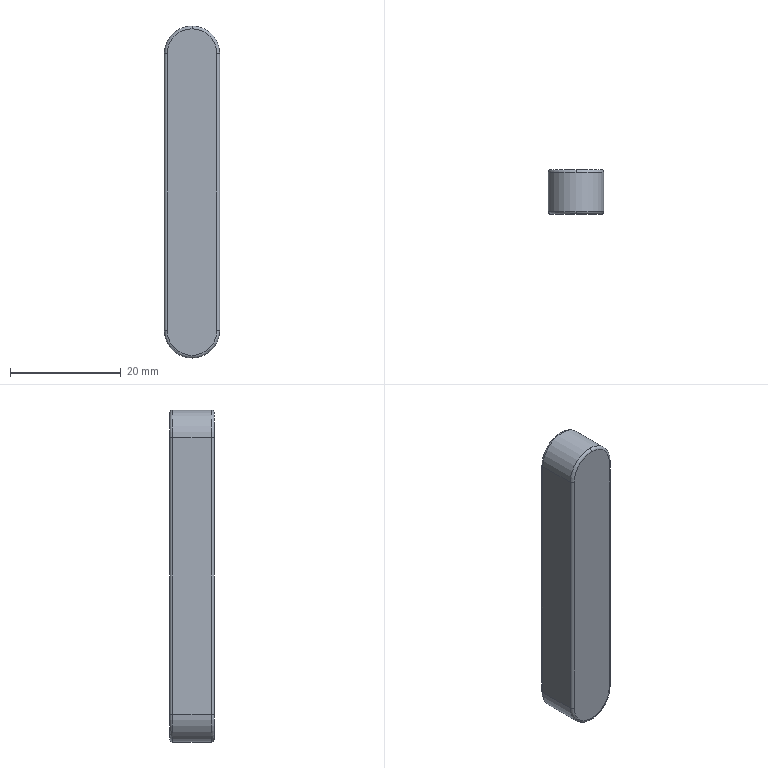Component | SolidWorks | 10X8X50ParallelKey-1 | 1 solid | 17 faces | box 10 x 8 x 60 mm | volume 4614 mm3 | cylinder 7 | torus 6 | plane 4 | commonest cylinder face diameters 1 x4 10 x3 | material AISI 1045 Steel, cold drawn
build123d program:
from build123d import *

# Parameters (mm, degrees)
BOSS_EXTRUDE1_DEPTH = 8
FILLET1_R           = 0.5


with BuildPart() as part:
    # Sketch1 → Boss-Extrude1 (new body)
    with BuildSketch(Plane.XY):
        with BuildLine():
            Line((-25, 5), (25, 5))
            ThreePointArc((25, 5), (30, 0), (25, -5))
            Line((25, -5), (-25, -5))
            ThreePointArc((-25, -5), (-30, 0), (-25, 5))
        make_face()
    extrude(amount=BOSS_EXTRUDE1_DEPTH)

    # Fillet1
    fillet1_edges = [part.edges().sort_by_distance(p)[0] for p in [
        (30, 0, 8),
        (0, 5, 8),
        (-30, 0, 8),
        (0, 5, 0),
        (30, 0, 0),
        (0, -5, 0),
        (-30, 0, 0),
        (0, -5, 8),
    ]]
    fillet(fillet1_edges, radius=FILLET1_R)


solid = part.part

# Placed as in the assembly
solid = solid.moved(Location((0, 18, 0), (90, 0, 90)))
STEP:
#1=CARTESIAN_POINT('',(0.,0.4134,1.181));
#2=VERTEX_POINT('',#1);
#3=CARTESIAN_POINT('',(0.1969,0.4134,0.9843));
#4=VERTEX_POINT('',#3);
#5=CARTESIAN_POINT('',(0.,0.4134,0.9843));
#6=DIRECTION('',(-0.,1.,0.));
#7=DIRECTION('',(0.,-0.,1.));
#8=AXIS2_PLACEMENT_3D('',#5,#6,#7);
#9=CIRCLE('',#8,0.1969);
#10=EDGE_CURVE('',#2,#4,#9,.T.);
#11=ORIENTED_EDGE('',*,*,#10,.F.);
#12=CARTESIAN_POINT('',(0.,0.3937,1.161));
#13=VERTEX_POINT('',#12);
#14=CARTESIAN_POINT('',(0.,0.4134,1.161));
#15=DIRECTION('',(1.,0.,0.));
#16=DIRECTION('',(-0.,1.,0.));
#17=AXIS2_PLACEMENT_3D('',#14,#15,#16);
#18=CIRCLE('',#17,0.01969);
#19=EDGE_CURVE('',#2,#13,#18,.T.);
#20=ORIENTED_EDGE('',*,*,#19,.T.);
#21=CARTESIAN_POINT('',(0.1772,0.3937,0.9843));
#22=VERTEX_POINT('',#21);
#23=CARTESIAN_POINT('',(0.,0.3937,0.9843));
#24=DIRECTION('',(0.,-1.,-0.));
#25=DIRECTION('',(0.,0.,1.));
#26=AXIS2_PLACEMENT_3D('',#23,#24,#25);
#27=CIRCLE('',#26,0.1772);
#28=EDGE_CURVE('',#22,#13,#27,.T.);
#29=ORIENTED_EDGE('',*,*,#28,.F.);
#30=CARTESIAN_POINT('',(0.1772,0.4134,0.9843));
#31=DIRECTION('',(0.,-0.,1.));
#32=DIRECTION('',(0.,1.,0.));
#33=AXIS2_PLACEMENT_3D('',#30,#31,#32);
#34=CIRCLE('',#33,0.01969);
#35=EDGE_CURVE('',#22,#4,#34,.T.);
#36=ORIENTED_EDGE('',*,*,#35,.T.);
#37=EDGE_LOOP('',(#11,#20,#29,#36));
#38=FACE_OUTER_BOUND('',#37,.T.);
#39=CARTESIAN_POINT('',(0.,0.4134,0.9843));
#40=DIRECTION('',(0.,-1.,-0.));
#41=DIRECTION('',(-0.,-0.,1.));
#42=AXIS2_PLACEMENT_3D('',#39,#40,#41);
#43=TOROIDAL_SURFACE('',#42,0.1772,0.01969);
#44=ADVANCED_FACE('',(#38),#43,.T.);
#45=CARTESIAN_POINT('',(0.,0.7087,1.161));
#46=VERTEX_POINT('',#45);
#47=CARTESIAN_POINT('',(0.1772,0.7087,0.9843));
#48=VERTEX_POINT('',#47);
#49=CARTESIAN_POINT('',(0.,0.7087,0.9843));
#50=DIRECTION('',(-0.,1.,0.));
#51=DIRECTION('',(0.,0.,1.));
#52=AXIS2_PLACEMENT_3D('',#49,#50,#51);
#53=CIRCLE('',#52,0.1772);
#54=EDGE_CURVE('',#46,#48,#53,.T.);
#55=ORIENTED_EDGE('',*,*,#54,.F.);
#56=CARTESIAN_POINT('',(0.,0.689,1.181));
#57=VERTEX_POINT('',#56);
#58=CARTESIAN_POINT('',(0.,0.689,1.161));
#59=DIRECTION('',(1.,0.,0.));
#60=DIRECTION('',(-0.,1.,0.));
#61=AXIS2_PLACEMENT_3D('',#58,#59,#60);
#62=CIRCLE('',#61,0.01969);
#63=EDGE_CURVE('',#46,#57,#62,.T.);
#64=ORIENTED_EDGE('',*,*,#63,.T.);
#65=CARTESIAN_POINT('',(0.1969,0.689,0.9843));
#66=VERTEX_POINT('',#65);
#67=CARTESIAN_POINT('',(0.,0.689,0.9843));
#68=DIRECTION('',(0.,-1.,-0.));
#69=DIRECTION('',(0.,0.,1.));
#70=AXIS2_PLACEMENT_3D('',#67,#68,#69);
#71=CIRCLE('',#70,0.1969);
#72=EDGE_CURVE('',#66,#57,#71,.T.);
#73=ORIENTED_EDGE('',*,*,#72,.F.);
#74=CARTESIAN_POINT('',(0.1772,0.689,0.9843));
#75=DIRECTION('',(0.,-0.,1.));
#76=DIRECTION('',(0.,1.,0.));
#77=AXIS2_PLACEMENT_3D('',#74,#75,#76);
#78=CIRCLE('',#77,0.01969);
#79=EDGE_CURVE('',#66,#48,#78,.T.);
#80=ORIENTED_EDGE('',*,*,#79,.T.);
#81=EDGE_LOOP('',(#55,#64,#73,#80));
#82=FACE_OUTER_BOUND('',#81,.T.);
#83=CARTESIAN_POINT('',(0.,0.689,0.9843));
#84=DIRECTION('',(0.,-1.,-0.));
#85=DIRECTION('',(0.,-0.,1.));
#86=AXIS2_PLACEMENT_3D('',#83,#84,#85);
#87=TOROIDAL_SURFACE('',#86,0.1772,0.01969);
#88=ADVANCED_FACE('',(#82),#87,.T.);
#89=CARTESIAN_POINT('',(0.1969,0.4134,-0.9843));
#90=VERTEX_POINT('',#89);
#91=CARTESIAN_POINT('',(0.,0.4134,-1.181));
#92=VERTEX_POINT('',#91);
#93=CARTESIAN_POINT('',(0.,0.4134,-0.9843));
#94=DIRECTION('',(-0.,1.,0.));
#95=DIRECTION('',(-0.,-0.,1.));
#96=AXIS2_PLACEMENT_3D('',#93,#94,#95);
#97=CIRCLE('',#96,0.1969);
#98=EDGE_CURVE('',#90,#92,#97,.T.);
#99=ORIENTED_EDGE('',*,*,#98,.T.);
#100=CARTESIAN_POINT('',(0.,0.689,-1.181));
#101=VERTEX_POINT('',#100);
#102=CARTESIAN_POINT('',(0.,0.3937,-1.181));
#103=DIRECTION('',(-0.,1.,0.));
#104=VECTOR('',#103,39.37);
#105=LINE('',#102,#104);
#106=EDGE_CURVE('',#92,#101,#105,.T.);
#107=ORIENTED_EDGE('',*,*,#106,.T.);
#108=CARTESIAN_POINT('',(0.1969,0.689,-0.9843));
#109=VERTEX_POINT('',#108);
#110=CARTESIAN_POINT('',(0.,0.689,-0.9843));
#111=DIRECTION('',(0.,-1.,-0.));
#112=DIRECTION('',(0.,0.,1.));
#113=AXIS2_PLACEMENT_3D('',#110,#111,#112);
#114=CIRCLE('',#113,0.1969);
#115=EDGE_CURVE('',#101,#109,#114,.T.);
#116=ORIENTED_EDGE('',*,*,#115,.T.);
#117=CARTESIAN_POINT('',(0.1969,0.3937,-0.9843));
#118=DIRECTION('',(-0.,1.,0.));
#119=VECTOR('',#118,39.37);
#120=LINE('',#117,#119);
#121=EDGE_CURVE('',#90,#109,#120,.T.);
#122=ORIENTED_EDGE('',*,*,#121,.F.);
#123=EDGE_LOOP('',(#99,#107,#116,#122));
#124=FACE_OUTER_BOUND('',#123,.T.);
#125=CARTESIAN_POINT('',(0.,0.3937,-0.9843));
#126=DIRECTION('',(-0.,1.,0.));
#127=DIRECTION('',(0.,0.,-1.));
#128=AXIS2_PLACEMENT_3D('',#125,#126,#127);
#129=CYLINDRICAL_SURFACE('',#128,0.1969);
#130=ADVANCED_FACE('',(#124),#129,.T.);
#131=ORIENTED_EDGE('',*,*,#106,.F.);
#132=CARTESIAN_POINT('',(-0.1969,0.4134,-0.9843));
#133=VERTEX_POINT('',#132);
#134=CARTESIAN_POINT('',(0.,0.4134,-0.9843));
#135=DIRECTION('',(-0.,1.,0.));
#136=DIRECTION('',(0.,-0.,1.));
#137=AXIS2_PLACEMENT_3D('',#134,#135,#136);
#138=CIRCLE('',#137,0.1969);
#139=EDGE_CURVE('',#92,#133,#138,.T.);
#140=ORIENTED_EDGE('',*,*,#139,.T.);
#141=CARTESIAN_POINT('',(-0.1969,0.689,-0.9843));
#142=VERTEX_POINT('',#141);
#143=CARTESIAN_POINT('',(-0.1969,0.3937,-0.9843));
#144=DIRECTION('',(-0.,1.,0.));
#145=VECTOR('',#144,39.37);
#146=LINE('',#143,#145);
#147=EDGE_CURVE('',#133,#142,#146,.T.);
#148=ORIENTED_EDGE('',*,*,#147,.T.);
#149=CARTESIAN_POINT('',(0.,0.689,-0.9843));
#150=DIRECTION('',(0.,-1.,-0.));
#151=DIRECTION('',(0.,0.,1.));
#152=AXIS2_PLACEMENT_3D('',#149,#150,#151);
#153=CIRCLE('',#152,0.1969);
#154=EDGE_CURVE('',#142,#101,#153,.T.);
#155=ORIENTED_EDGE('',*,*,#154,.T.);
#156=EDGE_LOOP('',(#131,#140,#148,#155));
#157=FACE_OUTER_BOUND('',#156,.T.);
#158=CARTESIAN_POINT('',(0.,0.3937,-0.9843));
#159=DIRECTION('',(-0.,1.,0.));
#160=DIRECTION('',(0.,0.,-1.));
#161=AXIS2_PLACEMENT_3D('',#158,#159,#160);
#162=CYLINDRICAL_SURFACE('',#161,0.1969);
#163=ADVANCED_FACE('',(#157),#162,.T.);
#164=ORIENTED_EDGE('',*,*,#121,.T.);
#165=CARTESIAN_POINT('',(0.1969,0.689,-0.9843));
#166=DIRECTION('',(0.,-0.,1.));
#167=VECTOR('',#166,39.37);
#168=LINE('',#165,#167);
#169=EDGE_CURVE('',#109,#66,#168,.T.);
#170=ORIENTED_EDGE('',*,*,#169,.T.);
#171=CARTESIAN_POINT('',(0.1969,0.3937,0.9843));
#172=DIRECTION('',(-0.,1.,0.));
#173=VECTOR('',#172,39.37);
#174=LINE('',#171,#173);
#175=EDGE_CURVE('',#4,#66,#174,.T.);
#176=ORIENTED_EDGE('',*,*,#175,.F.);
#177=CARTESIAN_POINT('',(0.1969,0.4134,-0.9843));
#178=DIRECTION('',(0.,0.,-1.));
#179=VECTOR('',#178,39.37);
#180=LINE('',#177,#179);
#181=EDGE_CURVE('',#4,#90,#180,.T.);
#182=ORIENTED_EDGE('',*,*,#181,.T.);
#183=EDGE_LOOP('',(#164,#170,#176,#182));
#184=FACE_OUTER_BOUND('',#183,.T.);
#185=CARTESIAN_POINT('',(0.1969,0.3937,-0.9843));
#186=DIRECTION('',(-1.,-0.,0.));
#187=DIRECTION('',(0.,-1.,-0.));
#188=AXIS2_PLACEMENT_3D('',#185,#186,#187);
#189=PLANE('',#188);
#190=ADVANCED_FACE('',(#184),#189,.F.);
#191=ORIENTED_EDGE('',*,*,#175,.T.);
#192=ORIENTED_EDGE('',*,*,#72,.T.);
#193=CARTESIAN_POINT('',(-0.1969,0.689,0.9843));
#194=VERTEX_POINT('',#193);
#195=CARTESIAN_POINT('',(0.,0.689,0.9843));
#196=DIRECTION('',(0.,-1.,-0.));
#197=DIRECTION('',(0.,0.,1.));
#198=AXIS2_PLACEMENT_3D('',#195,#196,#197);
#199=CIRCLE('',#198,0.1969);
#200=EDGE_CURVE('',#57,#194,#199,.T.);
#201=ORIENTED_EDGE('',*,*,#200,.T.);
#202=CARTESIAN_POINT('',(-0.1969,0.4134,0.9843));
#203=VERTEX_POINT('',#202);
#204=CARTESIAN_POINT('',(-0.1969,0.3937,0.9843));
#205=DIRECTION('',(-0.,1.,0.));
#206=VECTOR('',#205,39.37);
#207=LINE('',#204,#206);
#208=EDGE_CURVE('',#203,#194,#207,.T.);
#209=ORIENTED_EDGE('',*,*,#208,.F.);
#210=CARTESIAN_POINT('',(0.,0.4134,0.9843));
#211=DIRECTION('',(-0.,1.,0.));
#212=DIRECTION('',(-0.,-0.,1.));
#213=AXIS2_PLACEMENT_3D('',#210,#211,#212);
#214=CIRCLE('',#213,0.1969);
#215=EDGE_CURVE('',#203,#2,#214,.T.);
#216=ORIENTED_EDGE('',*,*,#215,.T.);
#217=ORIENTED_EDGE('',*,*,#10,.T.);
#218=EDGE_LOOP('',(#191,#192,#201,#209,#216,#217));
#219=FACE_OUTER_BOUND('',#218,.T.);
#220=CARTESIAN_POINT('',(0.,0.3937,0.9843));
#221=DIRECTION('',(-0.,1.,0.));
#222=DIRECTION('',(0.,0.,-1.));
#223=AXIS2_PLACEMENT_3D('',#220,#221,#222);
#224=CYLINDRICAL_SURFACE('',#223,0.1969);
#225=ADVANCED_FACE('',(#219),#224,.T.);
#226=ORIENTED_EDGE('',*,*,#208,.T.);
#227=CARTESIAN_POINT('',(-0.1969,0.689,-0.9843));
#228=DIRECTION('',(0.,0.,-1.));
#229=VECTOR('',#228,39.37);
#230=LINE('',#227,#229);
#231=EDGE_CURVE('',#194,#142,#230,.T.);
#232=ORIENTED_EDGE('',*,*,#231,.T.);
#233=ORIENTED_EDGE('',*,*,#147,.F.);
#234=CARTESIAN_POINT('',(-0.1969,0.4134,0.9843));
#235=DIRECTION('',(0.,-0.,1.));
#236=VECTOR('',#235,39.37);
#237=LINE('',#234,#236);
#238=EDGE_CURVE('',#133,#203,#237,.T.);
#239=ORIENTED_EDGE('',*,*,#238,.T.);
#240=EDGE_LOOP('',(#226,#232,#233,#239));
#241=FACE_OUTER_BOUND('',#240,.T.);
#242=CARTESIAN_POINT('',(-0.1969,0.3937,-0.9843));
#243=DIRECTION('',(1.,0.,-0.));
#244=DIRECTION('',(-0.,1.,0.));
#245=AXIS2_PLACEMENT_3D('',#242,#243,#244);
#246=PLANE('',#245);
#247=ADVANCED_FACE('',(#241),#246,.F.);
#248=ORIENTED_EDGE('',*,*,#28,.T.);
#249=CARTESIAN_POINT('',(-0.1772,0.3937,0.9843));
#250=VERTEX_POINT('',#249);
#251=CARTESIAN_POINT('',(0.,0.3937,0.9843));
#252=DIRECTION('',(0.,-1.,-0.));
#253=DIRECTION('',(0.,0.,1.));
#254=AXIS2_PLACEMENT_3D('',#251,#252,#253);
#255=CIRCLE('',#254,0.1772);
#256=EDGE_CURVE('',#13,#250,#255,.T.);
#257=ORIENTED_EDGE('',*,*,#256,.T.);
#258=CARTESIAN_POINT('',(-0.1772,0.3937,-0.9843));
#259=VERTEX_POINT('',#258);
#260=CARTESIAN_POINT('',(-0.1772,0.3937,-0.9843));
#261=DIRECTION('',(0.,0.,-1.));
#262=VECTOR('',#261,39.37);
#263=LINE('',#260,#262);
#264=EDGE_CURVE('',#250,#259,#263,.T.);
#265=ORIENTED_EDGE('',*,*,#264,.T.);
#266=CARTESIAN_POINT('',(0.1772,0.3937,-0.9843));
#267=VERTEX_POINT('',#266);
#268=CARTESIAN_POINT('',(0.,0.3937,-0.9843));
#269=DIRECTION('',(0.,-1.,-0.));
#270=DIRECTION('',(0.,0.,1.));
#271=AXIS2_PLACEMENT_3D('',#268,#269,#270);
#272=CIRCLE('',#271,0.1772);
#273=EDGE_CURVE('',#259,#267,#272,.T.);
#274=ORIENTED_EDGE('',*,*,#273,.T.);
#275=CARTESIAN_POINT('',(0.1772,0.3937,0.9843));
#276=DIRECTION('',(0.,-0.,1.));
#277=VECTOR('',#276,39.37);
#278=LINE('',#275,#277);
#279=EDGE_CURVE('',#267,#22,#278,.T.);
#280=ORIENTED_EDGE('',*,*,#279,.T.);
#281=EDGE_LOOP('',(#248,#257,#265,#274,#280));
#282=FACE_OUTER_BOUND('',#281,.T.);
#283=CARTESIAN_POINT('',(0.,0.3937,-0.9843));
#284=DIRECTION('',(0.,-1.,-0.));
#285=DIRECTION('',(0.,-0.,1.));
#286=AXIS2_PLACEMENT_3D('',#283,#284,#285);
#287=PLANE('',#286);
#288=ADVANCED_FACE('',(#282),#287,.T.);
#289=CARTESIAN_POINT('',(0.1772,0.7087,-0.9843));
#290=VERTEX_POINT('',#289);
#291=CARTESIAN_POINT('',(-0.1772,0.7087,-0.9843));
#292=VERTEX_POINT('',#291);
#293=CARTESIAN_POINT('',(0.,0.7087,-0.9843));
#294=DIRECTION('',(-0.,1.,0.));
#295=DIRECTION('',(-0.,0.,1.));
#296=AXIS2_PLACEMENT_3D('',#293,#294,#295);
#297=CIRCLE('',#296,0.1772);
#298=EDGE_CURVE('',#290,#292,#297,.T.);
#299=ORIENTED_EDGE('',*,*,#298,.T.);
#300=CARTESIAN_POINT('',(-0.1772,0.7087,0.9843));
#301=VERTEX_POINT('',#300);
#302=CARTESIAN_POINT('',(-0.1772,0.7087,-0.9843));
#303=DIRECTION('',(0.,-0.,1.));
#304=VECTOR('',#303,39.37);
#305=LINE('',#302,#304);
#306=EDGE_CURVE('',#292,#301,#305,.T.);
#307=ORIENTED_EDGE('',*,*,#306,.T.);
#308=CARTESIAN_POINT('',(0.,0.7087,0.9843));
#309=DIRECTION('',(-0.,1.,0.));
#310=DIRECTION('',(-0.,0.,1.));
#311=AXIS2_PLACEMENT_3D('',#308,#309,#310);
#312=CIRCLE('',#311,0.1772);
#313=EDGE_CURVE('',#301,#46,#312,.T.);
#314=ORIENTED_EDGE('',*,*,#313,.T.);
#315=ORIENTED_EDGE('',*,*,#54,.T.);
#316=CARTESIAN_POINT('',(0.1772,0.7087,-0.9843));
#317=DIRECTION('',(0.,0.,-1.));
#318=VECTOR('',#317,39.37);
#319=LINE('',#316,#318);
#320=EDGE_CURVE('',#48,#290,#319,.T.);
#321=ORIENTED_EDGE('',*,*,#320,.T.);
#322=EDGE_LOOP('',(#299,#307,#314,#315,#321));
#323=FACE_OUTER_BOUND('',#322,.T.);
#324=CARTESIAN_POINT('',(0.,0.7087,-0.9843));
#325=DIRECTION('',(0.,-1.,-0.));
#326=DIRECTION('',(0.,-0.,1.));
#327=AXIS2_PLACEMENT_3D('',#324,#325,#326);
#328=PLANE('',#327);
#329=ADVANCED_FACE('',(#323),#328,.F.);
#330=CARTESIAN_POINT('',(0.1772,0.689,-0.9843));
#331=DIRECTION('',(0.,0.,-1.));
#332=DIRECTION('',(0.,-1.,0.));
#333=AXIS2_PLACEMENT_3D('',#330,#331,#332);
#334=CIRCLE('',#333,0.01969);
#335=EDGE_CURVE('',#290,#109,#334,.T.);
#336=ORIENTED_EDGE('',*,*,#335,.F.);
#337=ORIENTED_EDGE('',*,*,#320,.F.);
#338=ORIENTED_EDGE('',*,*,#79,.F.);
#339=ORIENTED_EDGE('',*,*,#169,.F.);
#340=EDGE_LOOP('',(#336,#337,#338,#339));
#341=FACE_OUTER_BOUND('',#340,.T.);
#342=CARTESIAN_POINT('',(0.1772,0.689,-0.9843));
#343=DIRECTION('',(0.,-0.,1.));
#344=DIRECTION('',(0.,1.,0.));
#345=AXIS2_PLACEMENT_3D('',#342,#343,#344);
#346=CYLINDRICAL_SURFACE('',#345,0.01969);
#347=ADVANCED_FACE('',(#341),#346,.T.);
#348=ORIENTED_EDGE('',*,*,#63,.F.);
#349=ORIENTED_EDGE('',*,*,#313,.F.);
#350=CARTESIAN_POINT('',(-0.1772,0.689,0.9843));
#351=DIRECTION('',(0.,0.,-1.));
#352=DIRECTION('',(0.,-1.,0.));
#353=AXIS2_PLACEMENT_3D('',#350,#351,#352);
#354=CIRCLE('',#353,0.01969);
#355=EDGE_CURVE('',#194,#301,#354,.T.);
#356=ORIENTED_EDGE('',*,*,#355,.F.);
#357=ORIENTED_EDGE('',*,*,#200,.F.);
#358=EDGE_LOOP('',(#348,#349,#356,#357));
#359=FACE_OUTER_BOUND('',#358,.T.);
#360=CARTESIAN_POINT('',(0.,0.689,0.9843));
#361=DIRECTION('',(0.,-1.,-0.));
#362=DIRECTION('',(0.,-0.,1.));
#363=AXIS2_PLACEMENT_3D('',#360,#361,#362);
#364=TOROIDAL_SURFACE('',#363,0.1772,0.01969);
#365=ADVANCED_FACE('',(#359),#364,.T.);
#366=ORIENTED_EDGE('',*,*,#335,.T.);
#367=ORIENTED_EDGE('',*,*,#115,.F.);
#368=ORIENTED_EDGE('',*,*,#154,.F.);
#369=CARTESIAN_POINT('',(-0.1772,0.689,-0.9843));
#370=DIRECTION('',(0.,-0.,1.));
#371=DIRECTION('',(0.,1.,0.));
#372=AXIS2_PLACEMENT_3D('',#369,#370,#371);
#373=CIRCLE('',#372,0.01969);
#374=EDGE_CURVE('',#292,#142,#373,.T.);
#375=ORIENTED_EDGE('',*,*,#374,.F.);
#376=ORIENTED_EDGE('',*,*,#298,.F.);
#377=EDGE_LOOP('',(#366,#367,#368,#375,#376));
#378=FACE_OUTER_BOUND('',#377,.T.);
#379=CARTESIAN_POINT('',(0.,0.689,-0.9843));
#380=DIRECTION('',(0.,-1.,-0.));
#381=DIRECTION('',(0.,-0.,1.));
#382=AXIS2_PLACEMENT_3D('',#379,#380,#381);
#383=TOROIDAL_SURFACE('',#382,0.1772,0.01969);
#384=ADVANCED_FACE('',(#378),#383,.T.);
#385=ORIENTED_EDGE('',*,*,#355,.T.);
#386=ORIENTED_EDGE('',*,*,#306,.F.);
#387=ORIENTED_EDGE('',*,*,#374,.T.);
#388=ORIENTED_EDGE('',*,*,#231,.F.);
#389=EDGE_LOOP('',(#385,#386,#387,#388));
#390=FACE_OUTER_BOUND('',#389,.T.);
#391=CARTESIAN_POINT('',(-0.1772,0.689,-0.9843));
#392=DIRECTION('',(0.,0.,-1.));
#393=DIRECTION('',(0.,-1.,0.));
#394=AXIS2_PLACEMENT_3D('',#391,#392,#393);
#395=CYLINDRICAL_SURFACE('',#394,0.01969);
#396=ADVANCED_FACE('',(#390),#395,.T.);
#397=CARTESIAN_POINT('',(0.1772,0.4134,-0.9843));
#398=DIRECTION('',(0.,0.,-1.));
#399=DIRECTION('',(0.,-1.,0.));
#400=AXIS2_PLACEMENT_3D('',#397,#398,#399);
#401=CIRCLE('',#400,0.01969);
#402=EDGE_CURVE('',#90,#267,#401,.T.);
#403=ORIENTED_EDGE('',*,*,#402,.F.);
#404=ORIENTED_EDGE('',*,*,#181,.F.);
#405=ORIENTED_EDGE('',*,*,#35,.F.);
#406=ORIENTED_EDGE('',*,*,#279,.F.);
#407=EDGE_LOOP('',(#403,#404,#405,#406));
#408=FACE_OUTER_BOUND('',#407,.T.);
#409=CARTESIAN_POINT('',(0.1772,0.4134,-0.9843));
#410=DIRECTION('',(0.,0.,-1.));
#411=DIRECTION('',(0.,-1.,0.));
#412=AXIS2_PLACEMENT_3D('',#409,#410,#411);
#413=CYLINDRICAL_SURFACE('',#412,0.01969);
#414=ADVANCED_FACE('',(#408),#413,.T.);
#415=ORIENTED_EDGE('',*,*,#19,.F.);
#416=ORIENTED_EDGE('',*,*,#215,.F.);
#417=CARTESIAN_POINT('',(-0.1772,0.4134,0.9843));
#418=DIRECTION('',(0.,0.,-1.));
#419=DIRECTION('',(0.,-1.,0.));
#420=AXIS2_PLACEMENT_3D('',#417,#418,#419);
#421=CIRCLE('',#420,0.01969);
#422=EDGE_CURVE('',#250,#203,#421,.T.);
#423=ORIENTED_EDGE('',*,*,#422,.F.);
#424=ORIENTED_EDGE('',*,*,#256,.F.);
#425=EDGE_LOOP('',(#415,#416,#423,#424));
#426=FACE_OUTER_BOUND('',#425,.T.);
#427=CARTESIAN_POINT('',(0.,0.4134,0.9843));
#428=DIRECTION('',(0.,-1.,-0.));
#429=DIRECTION('',(-0.,-0.,1.));
#430=AXIS2_PLACEMENT_3D('',#427,#428,#429);
#431=TOROIDAL_SURFACE('',#430,0.1772,0.01969);
#432=ADVANCED_FACE('',(#426),#431,.T.);
#433=ORIENTED_EDGE('',*,*,#402,.T.);
#434=ORIENTED_EDGE('',*,*,#273,.F.);
#435=CARTESIAN_POINT('',(-0.1772,0.4134,-0.9843));
#436=DIRECTION('',(0.,-0.,1.));
#437=DIRECTION('',(0.,1.,0.));
#438=AXIS2_PLACEMENT_3D('',#435,#436,#437);
#439=CIRCLE('',#438,0.01969);
#440=EDGE_CURVE('',#133,#259,#439,.T.);
#441=ORIENTED_EDGE('',*,*,#440,.F.);
#442=ORIENTED_EDGE('',*,*,#139,.F.);
#443=ORIENTED_EDGE('',*,*,#98,.F.);
#444=EDGE_LOOP('',(#433,#434,#441,#442,#443));
#445=FACE_OUTER_BOUND('',#444,.T.);
#446=CARTESIAN_POINT('',(0.,0.4134,-0.9843));
#447=DIRECTION('',(0.,-1.,-0.));
#448=DIRECTION('',(-0.,-0.,1.));
#449=AXIS2_PLACEMENT_3D('',#446,#447,#448);
#450=TOROIDAL_SURFACE('',#449,0.1772,0.01969);
#451=ADVANCED_FACE('',(#445),#450,.T.);
#452=ORIENTED_EDGE('',*,*,#422,.T.);
#453=ORIENTED_EDGE('',*,*,#238,.F.);
#454=ORIENTED_EDGE('',*,*,#440,.T.);
#455=ORIENTED_EDGE('',*,*,#264,.F.);
#456=EDGE_LOOP('',(#452,#453,#454,#455));
#457=FACE_OUTER_BOUND('',#456,.T.);
#458=CARTESIAN_POINT('',(-0.1772,0.4134,-0.9843));
#459=DIRECTION('',(0.,-0.,1.));
#460=DIRECTION('',(0.,1.,0.));
#461=AXIS2_PLACEMENT_3D('',#458,#459,#460);
#462=CYLINDRICAL_SURFACE('',#461,0.01969);
#463=ADVANCED_FACE('',(#457),#462,.T.);
#464=CLOSED_SHELL('',(#44,#88,#130,#163,#190,#225,#247,#288,#329,#347,#365,#384,#396,#414,#432,#451,#463));
#465=MANIFOLD_SOLID_BREP('',#464);
#466=CARTESIAN_POINT('',(0.,0.,0.));
#467=DIRECTION('',(0.,0.,1.));
#468=DIRECTION('',(1.,0.,0.));
#469=AXIS2_PLACEMENT_3D('',#466,#467,#468);
#470=(LENGTH_UNIT()NAMED_UNIT(*)SI_UNIT($,.METRE.));
#471=LENGTH_MEASURE_WITH_UNIT(LENGTH_MEASURE(0.0254),#470);
#472=DIMENSIONAL_EXPONENTS(1.,0.,0.,0.,0.,0.,0.);
#473=(CONVERSION_BASED_UNIT('',#471)LENGTH_UNIT()NAMED_UNIT(#472));
#474=UNCERTAINTY_MEASURE_WITH_UNIT(LENGTH_MEASURE(0.00001),#473,'','');
#475=(NAMED_UNIT(*)PLANE_ANGLE_UNIT()SI_UNIT($,.RADIAN.));
#476=(NAMED_UNIT(*)SI_UNIT($,.STERADIAN.)SOLID_ANGLE_UNIT());
#477=(GEOMETRIC_REPRESENTATION_CONTEXT(3)GLOBAL_UNCERTAINTY_ASSIGNED_CONTEXT((#474))GLOBAL_UNIT_ASSIGNED_CONTEXT((#473,#475,#476))REPRESENTATION_CONTEXT('',''));
#478=ADVANCED_BREP_SHAPE_REPRESENTATION('',(#465,#469),#477);
#479=COLOUR_RGB('',0.7922,0.8196,0.9333);
#480=FILL_AREA_STYLE_COLOUR('',#479);
#481=FILL_AREA_STYLE('',(#480));
#482=SURFACE_STYLE_FILL_AREA(#481);
#483=SURFACE_SIDE_STYLE('',(#482));
#484=SURFACE_STYLE_USAGE(.BOTH.,#483);
#485=PRESENTATION_STYLE_ASSIGNMENT((#484));
#486=STYLED_ITEM('',(#485),#465);
#487=(LENGTH_UNIT()NAMED_UNIT(*)SI_UNIT($,.METRE.));
#488=LENGTH_MEASURE_WITH_UNIT(LENGTH_MEASURE(0.0254),#487);
#489=DIMENSIONAL_EXPONENTS(1.,0.,0.,0.,0.,0.,0.);
#490=(CONVERSION_BASED_UNIT('',#488)LENGTH_UNIT()NAMED_UNIT(#489));
#491=UNCERTAINTY_MEASURE_WITH_UNIT(LENGTH_MEASURE(0.00001),#490,'','');
#492=(NAMED_UNIT(*)PLANE_ANGLE_UNIT()SI_UNIT($,.RADIAN.));
#493=(NAMED_UNIT(*)SI_UNIT($,.STERADIAN.)SOLID_ANGLE_UNIT());
#494=(GEOMETRIC_REPRESENTATION_CONTEXT(3)GLOBAL_UNCERTAINTY_ASSIGNED_CONTEXT((#491))GLOBAL_UNIT_ASSIGNED_CONTEXT((#490,#492,#493))REPRESENTATION_CONTEXT('',''));
#495=MECHANICAL_DESIGN_GEOMETRIC_PRESENTATION_REPRESENTATION('',(#486),#494);
#496=PRESENTATION_LAYER_ASSIGNMENT('','',(#486));